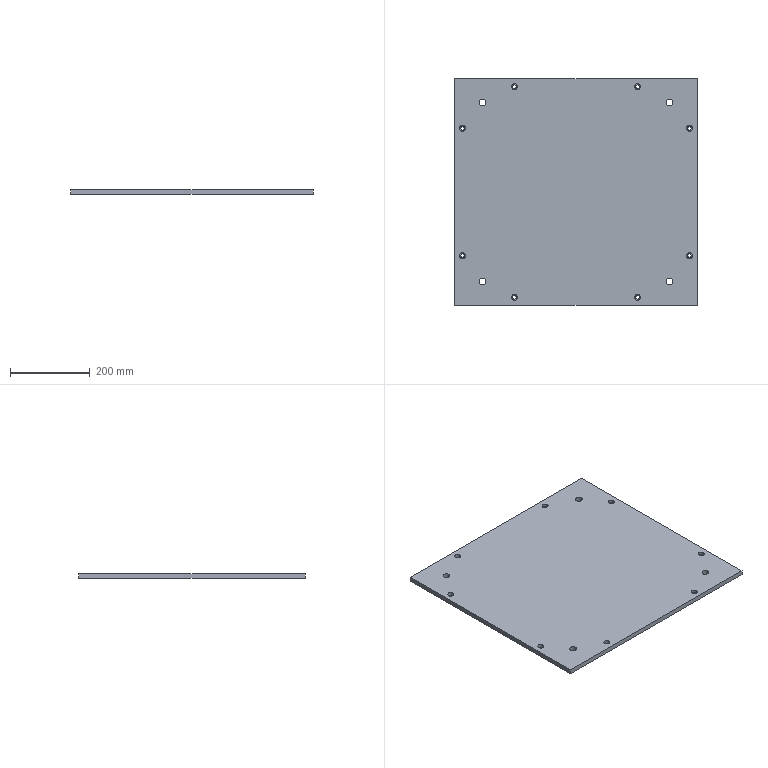Component | SolidWorks | CSFA2082 072-1 | 1 solid | 54 faces | box 610 x 570 x 12 mm | volume 4148159 mm3 | cylinder 40 | plane 14 | commonest cylinder face diameters 15 x16 9 x16 17 x8
build123d program:
from build123d import *

# Parameters (mm, degrees)
SKETCH1_W                                       = 610
SKETCH1_H                                       = 570
EXTRUDE1_DEPTH                                  = 12
F_17_0_17_DIAMETER_HOLE1_D                      = 17
F_17_0_17_DIAMETER_HOLE1_DEPTH                  = 71
F_17_0_17_DIAMETER_HOLE1_TIP                    = 5.107
M8_SOCKET_HEAD_CAP_SCREW_POST_HOLE1_D           = 9
M8_SOCKET_HEAD_CAP_SCREW_POST_HOLE1_CBORE_D     = 15
M8_SOCKET_HEAD_CAP_SCREW_POST_HOLE1_CBORE_DEPTH = 8


with BuildPart() as part:
    # Sketch1 → Extrude1 (new body)
    with BuildSketch(Plane.XY):
        Rectangle(SKETCH1_W, SKETCH1_H)
    extrude(amount=EXTRUDE1_DEPTH)

    # 17.0 _17_ Diameter Hole1
    with Locations(Plane.XY.offset(12)):
        with Locations((-235, 225), (-235, -225), (235, -225), (235, 225)):
            Hole(F_17_0_17_DIAMETER_HOLE1_D / 2, depth=F_17_0_17_DIAMETER_HOLE1_DEPTH)
            with Locations((0, 0, -(F_17_0_17_DIAMETER_HOLE1_DEPTH + F_17_0_17_DIAMETER_HOLE1_TIP / 2))):  # 118° drill point
                Cone(0, F_17_0_17_DIAMETER_HOLE1_D / 2, F_17_0_17_DIAMETER_HOLE1_TIP, mode=Mode.SUBTRACT)

    # M8 Socket Head Cap Screw Post Hole1 (through all)
    with Locations(Plane.XY.offset(12)):
        with Locations((-155, 265), (155, 265), (-155, -265), (155, -265), (-285, 160), (-285, -160), (285, 160), (285, -160)):
            CounterBoreHole(M8_SOCKET_HEAD_CAP_SCREW_POST_HOLE1_D / 2, M8_SOCKET_HEAD_CAP_SCREW_POST_HOLE1_CBORE_D / 2, M8_SOCKET_HEAD_CAP_SCREW_POST_HOLE1_CBORE_DEPTH)


solid = part.part

# Placed as in the assembly
solid = solid.moved(Location((-102.449, -16.176, 228), (0, 0, 0)))